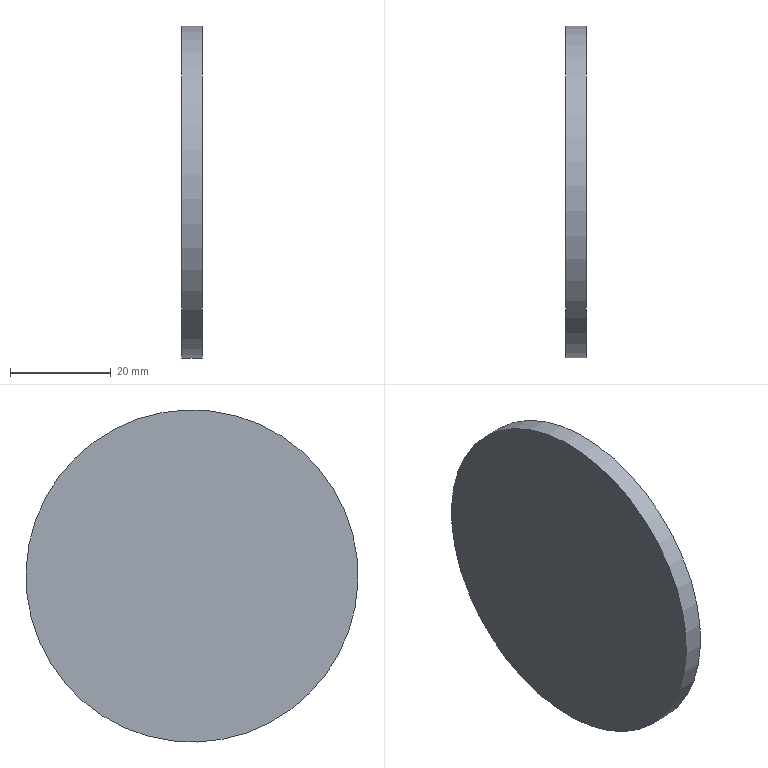Component | NX | DIAL1 | 1 solid | 3 faces | box 4 x 66 x 66 mm | volume 13685 mm3 | plane 2 | cylinder 1 | commonest cylinder face diameters 66 x1
STEP:
#1=CARTESIAN_POINT('',(0.,0.,0.));
#2=DIRECTION('',(0.,0.,1.));
#3=DIRECTION('',(1.,0.,0.));
#4=AXIS2_PLACEMENT_3D('',#1,#2,#3);
#5=CARTESIAN_POINT('',(-148.42,248.287,29.062));
#6=VERTEX_POINT('',#5);
#7=CARTESIAN_POINT('',(-148.42,281.257,30.472));
#8=DIRECTION('',(1.,0.,0.));
#9=DIRECTION('',(0.,-0.9991,-0.04272));
#10=AXIS2_PLACEMENT_3D('',#7,#8,#9);
#11=CIRCLE('',#10,33.);
#12=CARTESIAN_POINT('',(-148.42,281.257,30.472));
#13=DIRECTION('',(-1.,0.,0.));
#14=DIRECTION('',(0.,-0.9991,-0.04272));
#15=AXIS2_PLACEMENT_3D('',#12,#13,#14);
#16=PLANE('',#15);
#17=CARTESIAN_POINT('',(33.,0.));
#18=CARTESIAN_POINT('',(33.,-57.158));
#19=CARTESIAN_POINT('',(-16.5,-28.579));
#20=CARTESIAN_POINT('',(-66.,-0.));
#21=CARTESIAN_POINT('',(-16.5,28.579));
#22=CARTESIAN_POINT('',(33.,57.158));
#23=CARTESIAN_POINT('',(33.,0.));
#24=(BOUNDED_CURVE()B_SPLINE_CURVE(2,(#17,#18,#19,#20,#21,#22,#23),.UNSPECIFIED.,.T.,.F.)B_SPLINE_CURVE_WITH_KNOTS((1,2,2,2,2,1),(-2.094,0.,2.094,4.189,6.283,8.378),.UNSPECIFIED.)CURVE()GEOMETRIC_REPRESENTATION_ITEM()RATIONAL_B_SPLINE_CURVE((1.,0.5,1.,0.5,1.,0.5,1.))REPRESENTATION_ITEM(''));
#25=(GEOMETRIC_REPRESENTATION_CONTEXT(2)PARAMETRIC_REPRESENTATION_CONTEXT()REPRESENTATION_CONTEXT('',''));
#26=DEFINITIONAL_REPRESENTATION('',(#24),#25);
#27=PCURVE('',#16,#26);
#28=CARTESIAN_POINT('',(-144.42,281.257,30.472));
#29=DIRECTION('',(-1.,0.,0.));
#30=DIRECTION('',(0.,-0.9991,-0.04272));
#31=AXIS2_PLACEMENT_3D('',#28,#29,#30);
#32=CYLINDRICAL_SURFACE('',#31,33.);
#33=CARTESIAN_POINT('',(6.283,4.));
#34=DIRECTION('',(-1.,0.));
#35=VECTOR('',#34,1.);
#36=LINE('',#33,#35);
#37=(GEOMETRIC_REPRESENTATION_CONTEXT(2)PARAMETRIC_REPRESENTATION_CONTEXT()REPRESENTATION_CONTEXT('',''));
#38=DEFINITIONAL_REPRESENTATION('',(#36),#37);
#39=PCURVE('',#32,#38);
#40=SURFACE_CURVE('',#11,(#27,#39),.PCURVE_S1.);
#41=EDGE_CURVE('',#6,#6,#40,.T.);
#42=ORIENTED_EDGE('',*,*,#41,.F.);
#43=EDGE_LOOP('',(#42));
#44=FACE_BOUND('',#43,.T.);
#45=ADVANCED_FACE('',(#44),#16,.T.);
#46=CARTESIAN_POINT('',(-144.42,248.287,29.062));
#47=VERTEX_POINT('',#46);
#48=CARTESIAN_POINT('',(-144.42,281.257,30.472));
#49=DIRECTION('',(-1.,0.,0.));
#50=DIRECTION('',(0.,-0.9991,-0.04272));
#51=AXIS2_PLACEMENT_3D('',#48,#49,#50);
#52=CIRCLE('',#51,33.);
#53=CARTESIAN_POINT('',(-144.42,281.257,30.472));
#54=DIRECTION('',(1.,0.,0.));
#55=DIRECTION('',(0.,0.9991,0.04272));
#56=AXIS2_PLACEMENT_3D('',#53,#54,#55);
#57=PLANE('',#56);
#58=CARTESIAN_POINT('',(-33.,0.));
#59=CARTESIAN_POINT('',(-33.,57.158));
#60=CARTESIAN_POINT('',(16.5,28.579));
#61=CARTESIAN_POINT('',(66.,0.));
#62=CARTESIAN_POINT('',(16.5,-28.579));
#63=CARTESIAN_POINT('',(-33.,-57.158));
#64=CARTESIAN_POINT('',(-33.,0.));
#65=(BOUNDED_CURVE()B_SPLINE_CURVE(2,(#58,#59,#60,#61,#62,#63,#64),.UNSPECIFIED.,.T.,.F.)B_SPLINE_CURVE_WITH_KNOTS((1,2,2,2,2,1),(-2.094,0.,2.094,4.189,6.283,8.378),.UNSPECIFIED.)CURVE()GEOMETRIC_REPRESENTATION_ITEM()RATIONAL_B_SPLINE_CURVE((1.,0.5,1.,0.5,1.,0.5,1.))REPRESENTATION_ITEM(''));
#66=(GEOMETRIC_REPRESENTATION_CONTEXT(2)PARAMETRIC_REPRESENTATION_CONTEXT()REPRESENTATION_CONTEXT('',''));
#67=DEFINITIONAL_REPRESENTATION('',(#65),#66);
#68=PCURVE('',#57,#67);
#69=CARTESIAN_POINT('',(0.,0.));
#70=DIRECTION('',(1.,0.));
#71=VECTOR('',#70,1.);
#72=LINE('',#69,#71);
#73=(GEOMETRIC_REPRESENTATION_CONTEXT(2)PARAMETRIC_REPRESENTATION_CONTEXT()REPRESENTATION_CONTEXT('',''));
#74=DEFINITIONAL_REPRESENTATION('',(#72),#73);
#75=PCURVE('',#32,#74);
#76=SURFACE_CURVE('',#52,(#68,#75),.PCURVE_S1.);
#77=EDGE_CURVE('',#47,#47,#76,.T.);
#78=ORIENTED_EDGE('',*,*,#77,.F.);
#79=EDGE_LOOP('',(#78));
#80=FACE_BOUND('',#79,.T.);
#81=ADVANCED_FACE('',(#80),#57,.T.);
#82=ORIENTED_EDGE('',*,*,#41,.T.);
#83=CARTESIAN_POINT('',(-144.42,248.287,29.062));
#84=CARTESIAN_POINT('',(-148.42,248.287,29.062));
#85=B_SPLINE_CURVE_WITH_KNOTS('',1,(#83,#84),.UNSPECIFIED.,.F.,.F.,(2,2),(0.,4.),.PIECEWISE_BEZIER_KNOTS.);
#86=CARTESIAN_POINT('',(0.,0.));
#87=DIRECTION('',(0.,1.));
#88=VECTOR('',#87,1.);
#89=LINE('',#86,#88);
#90=(GEOMETRIC_REPRESENTATION_CONTEXT(2)PARAMETRIC_REPRESENTATION_CONTEXT()REPRESENTATION_CONTEXT('',''));
#91=DEFINITIONAL_REPRESENTATION('',(#89),#90);
#92=PCURVE('',#32,#91);
#93=CARTESIAN_POINT('',(6.283,0.));
#94=DIRECTION('',(0.,1.));
#95=VECTOR('',#94,1.);
#96=LINE('',#93,#95);
#97=(GEOMETRIC_REPRESENTATION_CONTEXT(2)PARAMETRIC_REPRESENTATION_CONTEXT()REPRESENTATION_CONTEXT('',''));
#98=DEFINITIONAL_REPRESENTATION('',(#96),#97);
#99=PCURVE('',#32,#98);
#100=SEAM_CURVE('',#85,(#92,#99),.PCURVE_S1.);
#101=EDGE_CURVE('',#47,#6,#100,.T.);
#102=ORIENTED_EDGE('',*,*,#101,.F.);
#103=ORIENTED_EDGE('',*,*,#77,.T.);
#104=ORIENTED_EDGE('',*,*,#101,.T.);
#105=EDGE_LOOP('',(#82,#102,#103,#104));
#106=FACE_BOUND('',#105,.T.);
#107=ADVANCED_FACE('',(#106),#32,.T.);
#108=CLOSED_SHELL('',(#45,#81,#107));
#109=MANIFOLD_SOLID_BREP('',#108);
#110=(LENGTH_UNIT()NAMED_UNIT(*)SI_UNIT(.MILLI.,.METRE.));
#111=UNCERTAINTY_MEASURE_WITH_UNIT(LENGTH_MEASURE(0.00001),#110,'','');
#112=(NAMED_UNIT(*)PLANE_ANGLE_UNIT()SI_UNIT($,.RADIAN.));
#113=(NAMED_UNIT(*)SI_UNIT($,.STERADIAN.)SOLID_ANGLE_UNIT());
#114=(GEOMETRIC_REPRESENTATION_CONTEXT(3)GLOBAL_UNCERTAINTY_ASSIGNED_CONTEXT((#111))GLOBAL_UNIT_ASSIGNED_CONTEXT((#110,#112,#113))REPRESENTATION_CONTEXT('',''));
#115=ADVANCED_BREP_SHAPE_REPRESENTATION('',(#4,#109),#114);